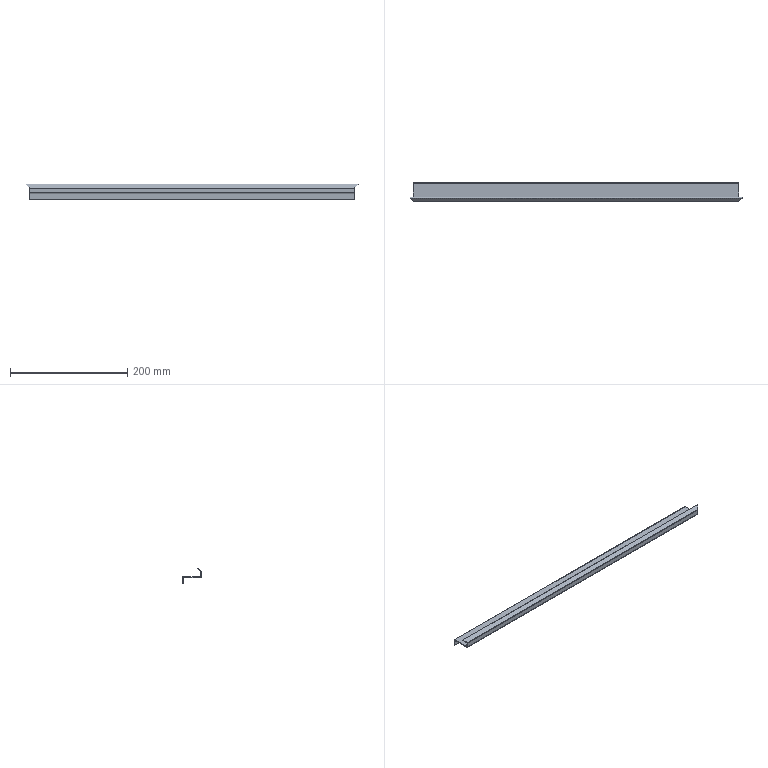Component | SolidWorks | UpperBeam-1 | 1 solid | 30 faces | box 566.33 x 32 x 26.16 mm | volume 48106 mm3 | plane 22 | cylinder 6 | spline 2 | commonest cylinder face diameters 3.2 x3 0.2 x3
STEP:
#1=COLOUR_RGB('',0.7922,0.8196,0.9333);
#2=FILL_AREA_STYLE_COLOUR('',#1);
#3=FILL_AREA_STYLE('',(#2));
#4=SURFACE_STYLE_FILL_AREA(#3);
#5=SURFACE_SIDE_STYLE('',(#4));
#6=SURFACE_STYLE_USAGE(.BOTH.,#5);
#7=PRESENTATION_STYLE_ASSIGNMENT((#6));
#8=CARTESIAN_POINT('',(9.198,12.971,37.604));
#9=VERTEX_POINT('',#8);
#10=CARTESIAN_POINT('',(9.198,14.105,37.604));
#11=VERTEX_POINT('',#10);
#12=CARTESIAN_POINT('',(9.198,12.908,37.604));
#13=DIRECTION('',(0.,1.,0.));
#14=VECTOR('',#13,39.37);
#15=LINE('',#12,#14);
#16=EDGE_CURVE('',#9,#11,#15,.T.);
#17=ORIENTED_EDGE('',*,*,#16,.T.);
#18=CARTESIAN_POINT('',(9.198,14.105,37.663));
#19=VERTEX_POINT('',#18);
#20=CARTESIAN_POINT('',(9.198,14.105,37.604));
#21=DIRECTION('',(0.,0.,1.));
#22=VECTOR('',#21,39.37);
#23=LINE('',#20,#22);
#24=EDGE_CURVE('',#11,#19,#23,.T.);
#25=ORIENTED_EDGE('',*,*,#24,.T.);
#26=CARTESIAN_POINT('',(9.198,12.971,37.663));
#27=VERTEX_POINT('',#26);
#28=CARTESIAN_POINT('',(9.198,12.908,37.663));
#29=DIRECTION('',(0.,1.,0.));
#30=VECTOR('',#29,39.37);
#31=LINE('',#28,#30);
#32=EDGE_CURVE('',#27,#19,#31,.T.);
#33=ORIENTED_EDGE('',*,*,#32,.F.);
#34=CARTESIAN_POINT('',(9.198,12.971,37.663));
#35=DIRECTION('',(0.,0.,-1.));
#36=VECTOR('',#35,39.37);
#37=LINE('',#34,#36);
#38=EDGE_CURVE('',#27,#9,#37,.T.);
#39=ORIENTED_EDGE('',*,*,#38,.T.);
#40=EDGE_LOOP('',(#17,#25,#33,#39));
#41=FACE_OUTER_BOUND('',#40,.T.);
#42=CARTESIAN_POINT('',(9.198,12.908,37.604));
#43=DIRECTION('',(1.,0.,0.));
#44=DIRECTION('',(0.,0.,-1.));
#45=AXIS2_PLACEMENT_3D('',#42,#43,#44);
#46=PLANE('',#45);
#47=ADVANCED_FACE('',(#41),#46,.T.);
#48=CARTESIAN_POINT('',(-12.691,14.105,37.604));
#49=VERTEX_POINT('',#48);
#50=CARTESIAN_POINT('',(-12.691,12.971,37.604));
#51=VERTEX_POINT('',#50);
#52=CARTESIAN_POINT('',(-12.691,12.908,37.604));
#53=DIRECTION('',(0.,-1.,0.));
#54=VECTOR('',#53,39.37);
#55=LINE('',#52,#54);
#56=EDGE_CURVE('',#49,#51,#55,.T.);
#57=ORIENTED_EDGE('',*,*,#56,.F.);
#58=CARTESIAN_POINT('',(9.198,14.105,37.604));
#59=DIRECTION('',(-1.,0.,0.));
#60=VECTOR('',#59,39.37);
#61=LINE('',#58,#60);
#62=EDGE_CURVE('',#11,#49,#61,.T.);
#63=ORIENTED_EDGE('',*,*,#62,.F.);
#64=ORIENTED_EDGE('',*,*,#16,.F.);
#65=CARTESIAN_POINT('',(9.198,12.971,37.604));
#66=DIRECTION('',(-1.,0.,0.));
#67=VECTOR('',#66,39.37);
#68=LINE('',#65,#67);
#69=EDGE_CURVE('',#9,#51,#68,.T.);
#70=ORIENTED_EDGE('',*,*,#69,.T.);
#71=EDGE_LOOP('',(#57,#63,#64,#70));
#72=FACE_OUTER_BOUND('',#71,.T.);
#73=CARTESIAN_POINT('',(-1.746,13.538,37.604));
#74=DIRECTION('',(0.,0.,-1.));
#75=DIRECTION('',(-1.,0.,0.));
#76=AXIS2_PLACEMENT_3D('',#73,#74,#75);
#77=PLANE('',#76);
#78=ADVANCED_FACE('',(#72),#77,.T.);
#79=CARTESIAN_POINT('',(-12.691,14.105,37.663));
#80=VERTEX_POINT('',#79);
#81=CARTESIAN_POINT('',(9.198,14.105,37.663));
#82=DIRECTION('',(-1.,0.,0.));
#83=VECTOR('',#82,39.37);
#84=LINE('',#81,#83);
#85=EDGE_CURVE('',#19,#80,#84,.T.);
#86=ORIENTED_EDGE('',*,*,#85,.T.);
#87=CARTESIAN_POINT('',(-12.691,12.971,37.663));
#88=VERTEX_POINT('',#87);
#89=CARTESIAN_POINT('',(-12.691,12.908,37.663));
#90=DIRECTION('',(0.,-1.,0.));
#91=VECTOR('',#90,39.37);
#92=LINE('',#89,#91);
#93=EDGE_CURVE('',#80,#88,#92,.T.);
#94=ORIENTED_EDGE('',*,*,#93,.T.);
#95=CARTESIAN_POINT('',(9.198,12.971,37.663));
#96=DIRECTION('',(-1.,0.,0.));
#97=VECTOR('',#96,39.37);
#98=LINE('',#95,#97);
#99=EDGE_CURVE('',#27,#88,#98,.T.);
#100=ORIENTED_EDGE('',*,*,#99,.F.);
#101=ORIENTED_EDGE('',*,*,#32,.T.);
#102=EDGE_LOOP('',(#86,#94,#100,#101));
#103=FACE_OUTER_BOUND('',#102,.T.);
#104=CARTESIAN_POINT('',(-1.746,13.538,37.663));
#105=DIRECTION('',(0.,0.,-1.));
#106=DIRECTION('',(-1.,0.,0.));
#107=AXIS2_PLACEMENT_3D('',#104,#105,#106);
#108=PLANE('',#107);
#109=ADVANCED_FACE('',(#103),#108,.F.);
#110=CARTESIAN_POINT('',(9.198,12.967,37.971));
#111=VERTEX_POINT('',#110);
#112=CARTESIAN_POINT('',(9.198,12.908,37.971));
#113=VERTEX_POINT('',#112);
#114=CARTESIAN_POINT('',(9.198,12.967,37.971));
#115=DIRECTION('',(0.,-1.,0.));
#116=VECTOR('',#115,39.37);
#117=LINE('',#114,#116);
#118=EDGE_CURVE('',#111,#113,#117,.T.);
#119=ORIENTED_EDGE('',*,*,#118,.T.);
#120=CARTESIAN_POINT('',(9.198,12.908,37.667));
#121=VERTEX_POINT('',#120);
#122=CARTESIAN_POINT('',(9.198,12.908,37.663));
#123=DIRECTION('',(0.,-0.,1.));
#124=VECTOR('',#123,39.37);
#125=LINE('',#122,#124);
#126=EDGE_CURVE('',#121,#113,#125,.T.);
#127=ORIENTED_EDGE('',*,*,#126,.F.);
#128=CARTESIAN_POINT('',(9.198,12.967,37.667));
#129=VERTEX_POINT('',#128);
#130=CARTESIAN_POINT('',(9.198,12.967,37.667));
#131=DIRECTION('',(0.,-1.,-0.));
#132=VECTOR('',#131,39.37);
#133=LINE('',#130,#132);
#134=EDGE_CURVE('',#129,#121,#133,.T.);
#135=ORIENTED_EDGE('',*,*,#134,.F.);
#136=CARTESIAN_POINT('',(9.198,12.967,37.998));
#137=DIRECTION('',(0.,-0.,1.));
#138=VECTOR('',#137,39.37);
#139=LINE('',#136,#138);
#140=EDGE_CURVE('',#129,#111,#139,.T.);
#141=ORIENTED_EDGE('',*,*,#140,.T.);
#142=EDGE_LOOP('',(#119,#127,#135,#141));
#143=FACE_OUTER_BOUND('',#142,.T.);
#144=CARTESIAN_POINT('',(9.198,12.908,37.998));
#145=DIRECTION('',(-1.,0.,0.));
#146=DIRECTION('',(0.,0.,1.));
#147=AXIS2_PLACEMENT_3D('',#144,#145,#146);
#148=PLANE('',#147);
#149=ADVANCED_FACE('',(#143),#148,.F.);
#150=CARTESIAN_POINT('',(-12.691,12.967,37.971));
#151=VERTEX_POINT('',#150);
#152=CARTESIAN_POINT('',(-12.691,12.908,37.971));
#153=VERTEX_POINT('',#152);
#154=CARTESIAN_POINT('',(-12.691,12.967,37.971));
#155=DIRECTION('',(0.,-1.,0.));
#156=VECTOR('',#155,39.37);
#157=LINE('',#154,#156);
#158=EDGE_CURVE('',#151,#153,#157,.T.);
#159=ORIENTED_EDGE('',*,*,#158,.F.);
#160=CARTESIAN_POINT('',(-12.691,12.967,37.667));
#161=VERTEX_POINT('',#160);
#162=CARTESIAN_POINT('',(-12.691,12.967,37.663));
#163=DIRECTION('',(0.,0.,-1.));
#164=VECTOR('',#163,39.37);
#165=LINE('',#162,#164);
#166=EDGE_CURVE('',#151,#161,#165,.T.);
#167=ORIENTED_EDGE('',*,*,#166,.T.);
#168=CARTESIAN_POINT('',(-12.691,12.908,37.667));
#169=VERTEX_POINT('',#168);
#170=CARTESIAN_POINT('',(-12.691,12.908,37.667));
#171=DIRECTION('',(0.,-1.,-0.));
#172=VECTOR('',#171,39.37);
#173=LINE('',#170,#172);
#174=EDGE_CURVE('',#161,#169,#173,.T.);
#175=ORIENTED_EDGE('',*,*,#174,.T.);
#176=CARTESIAN_POINT('',(-12.691,12.908,37.663));
#177=DIRECTION('',(0.,0.,-1.));
#178=VECTOR('',#177,39.37);
#179=LINE('',#176,#178);
#180=EDGE_CURVE('',#153,#169,#179,.T.);
#181=ORIENTED_EDGE('',*,*,#180,.F.);
#182=EDGE_LOOP('',(#159,#167,#175,#181));
#183=FACE_OUTER_BOUND('',#182,.T.);
#184=CARTESIAN_POINT('',(-12.691,12.908,37.663));
#185=DIRECTION('',(1.,0.,0.));
#186=DIRECTION('',(0.,0.,-1.));
#187=AXIS2_PLACEMENT_3D('',#184,#185,#186);
#188=PLANE('',#187);
#189=ADVANCED_FACE('',(#183),#188,.F.);
#190=CARTESIAN_POINT('',(9.2,12.908,37.971));
#191=DIRECTION('',(-1.,0.,0.));
#192=VECTOR('',#191,39.37);
#193=LINE('',#190,#192);
#194=EDGE_CURVE('',#113,#153,#193,.T.);
#195=ORIENTED_EDGE('',*,*,#194,.T.);
#196=ORIENTED_EDGE('',*,*,#180,.T.);
#197=CARTESIAN_POINT('',(-12.691,12.908,37.667));
#198=DIRECTION('',(-1.,-0.,0.));
#199=VECTOR('',#198,39.37);
#200=LINE('',#197,#199);
#201=EDGE_CURVE('',#121,#169,#200,.T.);
#202=ORIENTED_EDGE('',*,*,#201,.F.);
#203=ORIENTED_EDGE('',*,*,#126,.T.);
#204=EDGE_LOOP('',(#195,#196,#202,#203));
#205=FACE_OUTER_BOUND('',#204,.T.);
#206=CARTESIAN_POINT('',(-1.746,12.908,37.663));
#207=DIRECTION('',(0.,1.,0.));
#208=DIRECTION('',(0.,-0.,1.));
#209=AXIS2_PLACEMENT_3D('',#206,#207,#208);
#210=PLANE('',#209);
#211=ADVANCED_FACE('',(#205),#210,.F.);
#212=ORIENTED_EDGE('',*,*,#166,.F.);
#213=CARTESIAN_POINT('',(9.2,12.967,37.971));
#214=DIRECTION('',(-1.,0.,0.));
#215=VECTOR('',#214,39.37);
#216=LINE('',#213,#215);
#217=EDGE_CURVE('',#111,#151,#216,.T.);
#218=ORIENTED_EDGE('',*,*,#217,.F.);
#219=ORIENTED_EDGE('',*,*,#140,.F.);
#220=CARTESIAN_POINT('',(-12.691,12.967,37.667));
#221=DIRECTION('',(1.,0.,-0.));
#222=VECTOR('',#221,39.37);
#223=LINE('',#220,#222);
#224=EDGE_CURVE('',#161,#129,#223,.T.);
#225=ORIENTED_EDGE('',*,*,#224,.F.);
#226=EDGE_LOOP('',(#212,#218,#219,#225));
#227=FACE_OUTER_BOUND('',#226,.T.);
#228=CARTESIAN_POINT('',(-1.746,12.967,37.663));
#229=DIRECTION('',(0.,1.,0.));
#230=DIRECTION('',(0.,-0.,1.));
#231=AXIS2_PLACEMENT_3D('',#228,#229,#230);
#232=PLANE('',#231);
#233=ADVANCED_FACE('',(#227),#232,.T.);
#234=CARTESIAN_POINT('',(-12.691,14.105,37.604));
#235=DIRECTION('',(0.,0.,1.));
#236=VECTOR('',#235,39.37);
#237=LINE('',#234,#236);
#238=EDGE_CURVE('',#49,#80,#237,.T.);
#239=ORIENTED_EDGE('',*,*,#238,.F.);
#240=ORIENTED_EDGE('',*,*,#56,.T.);
#241=CARTESIAN_POINT('',(-12.691,12.971,37.663));
#242=DIRECTION('',(0.,0.,-1.));
#243=VECTOR('',#242,39.37);
#244=LINE('',#241,#243);
#245=EDGE_CURVE('',#88,#51,#244,.T.);
#246=ORIENTED_EDGE('',*,*,#245,.F.);
#247=ORIENTED_EDGE('',*,*,#93,.F.);
#248=EDGE_LOOP('',(#239,#240,#246,#247));
#249=FACE_OUTER_BOUND('',#248,.T.);
#250=CARTESIAN_POINT('',(-12.691,12.908,37.604));
#251=DIRECTION('',(-1.,0.,0.));
#252=DIRECTION('',(0.,0.,1.));
#253=AXIS2_PLACEMENT_3D('',#250,#251,#252);
#254=PLANE('',#253);
#255=ADVANCED_FACE('',(#249),#254,.T.);
#256=ORIENTED_EDGE('',*,*,#174,.F.);
#257=CARTESIAN_POINT('',(-12.691,12.971,37.667));
#258=DIRECTION('',(-1.,0.,0.));
#259=DIRECTION('',(0.,0.,-1.));
#260=AXIS2_PLACEMENT_3D('',#257,#258,#259);
#261=CIRCLE('',#260,0.003937);
#262=EDGE_CURVE('',#88,#161,#261,.T.);
#263=ORIENTED_EDGE('',*,*,#262,.F.);
#264=ORIENTED_EDGE('',*,*,#245,.T.);
#265=CARTESIAN_POINT('',(-12.691,12.971,37.667));
#266=DIRECTION('',(-1.,0.,0.));
#267=DIRECTION('',(0.,0.,-1.));
#268=AXIS2_PLACEMENT_3D('',#265,#266,#267);
#269=CIRCLE('',#268,0.06299);
#270=EDGE_CURVE('',#51,#169,#269,.T.);
#271=ORIENTED_EDGE('',*,*,#270,.T.);
#272=EDGE_LOOP('',(#256,#263,#264,#271));
#273=FACE_OUTER_BOUND('',#272,.T.);
#274=CARTESIAN_POINT('',(-12.691,12.971,37.667));
#275=DIRECTION('',(-1.,0.,0.));
#276=DIRECTION('',(0.,0.,1.));
#277=AXIS2_PLACEMENT_3D('',#274,#275,#276);
#278=PLANE('',#277);
#279=ADVANCED_FACE('',(#273),#278,.T.);
#280=CARTESIAN_POINT('',(9.198,12.971,37.667));
#281=DIRECTION('',(1.,0.,0.));
#282=DIRECTION('',(0.,0.,-1.));
#283=AXIS2_PLACEMENT_3D('',#280,#281,#282);
#284=CIRCLE('',#283,0.003937);
#285=EDGE_CURVE('',#129,#27,#284,.T.);
#286=ORIENTED_EDGE('',*,*,#285,.F.);
#287=ORIENTED_EDGE('',*,*,#134,.T.);
#288=CARTESIAN_POINT('',(9.198,12.971,37.667));
#289=DIRECTION('',(1.,0.,0.));
#290=DIRECTION('',(0.,0.,-1.));
#291=AXIS2_PLACEMENT_3D('',#288,#289,#290);
#292=CIRCLE('',#291,0.06299);
#293=EDGE_CURVE('',#121,#9,#292,.T.);
#294=ORIENTED_EDGE('',*,*,#293,.T.);
#295=ORIENTED_EDGE('',*,*,#38,.F.);
#296=EDGE_LOOP('',(#286,#287,#294,#295));
#297=FACE_OUTER_BOUND('',#296,.T.);
#298=CARTESIAN_POINT('',(9.198,12.971,37.667));
#299=DIRECTION('',(-1.,0.,0.));
#300=DIRECTION('',(0.,0.,1.));
#301=AXIS2_PLACEMENT_3D('',#298,#299,#300);
#302=PLANE('',#301);
#303=ADVANCED_FACE('',(#297),#302,.F.);
#304=ORIENTED_EDGE('',*,*,#69,.F.);
#305=ORIENTED_EDGE('',*,*,#293,.F.);
#306=ORIENTED_EDGE('',*,*,#201,.T.);
#307=ORIENTED_EDGE('',*,*,#270,.F.);
#308=EDGE_LOOP('',(#304,#305,#306,#307));
#309=FACE_OUTER_BOUND('',#308,.T.);
#310=CARTESIAN_POINT('',(9.198,12.971,37.667));
#311=DIRECTION('',(1.,0.,0.));
#312=DIRECTION('',(0.,-1.,0.));
#313=AXIS2_PLACEMENT_3D('',#310,#311,#312);
#314=CYLINDRICAL_SURFACE('',#313,0.06299);
#315=ADVANCED_FACE('',(#309),#314,.T.);
#316=ORIENTED_EDGE('',*,*,#99,.T.);
#317=ORIENTED_EDGE('',*,*,#262,.T.);
#318=ORIENTED_EDGE('',*,*,#224,.T.);
#319=ORIENTED_EDGE('',*,*,#285,.T.);
#320=EDGE_LOOP('',(#316,#317,#318,#319));
#321=FACE_OUTER_BOUND('',#320,.T.);
#322=CARTESIAN_POINT('',(9.198,12.971,37.667));
#323=DIRECTION('',(1.,0.,0.));
#324=DIRECTION('',(0.,-1.,0.));
#325=AXIS2_PLACEMENT_3D('',#322,#323,#324);
#326=CYLINDRICAL_SURFACE('',#325,0.003937);
#327=ADVANCED_FACE('',(#321),#326,.F.);
#328=CARTESIAN_POINT('',(-12.692,12.968,37.974));
#329=VERTEX_POINT('',#328);
#330=CARTESIAN_POINT('',(-12.692,12.927,38.016));
#331=VERTEX_POINT('',#330);
#332=CARTESIAN_POINT('',(-12.692,12.927,38.016));
#333=DIRECTION('',(0.,-0.7071,0.7071));
#334=VECTOR('',#333,39.37);
#335=LINE('',#332,#334);
#336=EDGE_CURVE('',#329,#331,#335,.T.);
#337=ORIENTED_EDGE('',*,*,#336,.F.);
#338=CARTESIAN_POINT('',(-12.691,12.967,37.971));
#339=CARTESIAN_POINT('',(-12.692,12.967,37.972));
#340=CARTESIAN_POINT('',(-12.692,12.968,37.973));
#341=CARTESIAN_POINT('',(-12.692,12.968,37.974));
#342=B_SPLINE_CURVE_WITH_KNOTS('',3,(#338,#339,#340,#341),.UNSPECIFIED.,.F.,.F.,(4,4),(0.,1.),.UNSPECIFIED.);
#343=EDGE_CURVE('',#151,#329,#342,.T.);
#344=ORIENTED_EDGE('',*,*,#343,.F.);
#345=ORIENTED_EDGE('',*,*,#158,.T.);
#346=CARTESIAN_POINT('',(-12.691,12.908,37.971));
#347=CARTESIAN_POINT('',(-12.692,12.908,37.98));
#348=CARTESIAN_POINT('',(-12.692,12.91,37.988));
#349=CARTESIAN_POINT('',(-12.692,12.916,38.003));
#350=CARTESIAN_POINT('',(-12.692,12.921,38.01));
#351=CARTESIAN_POINT('',(-12.692,12.927,38.016));
#352=B_SPLINE_CURVE_WITH_KNOTS('',3,(#346,#347,#348,#349,#350,#351),.UNSPECIFIED.,.F.,.F.,(4,2,4),(0.,0.5,1.),.UNSPECIFIED.);
#353=EDGE_CURVE('',#153,#331,#352,.T.);
#354=ORIENTED_EDGE('',*,*,#353,.T.);
#355=EDGE_LOOP('',(#337,#344,#345,#354));
#356=FACE_OUTER_BOUND('',#355,.T.);
#357=CARTESIAN_POINT('',(-12.691,12.908,37.971));
#358=CARTESIAN_POINT('',(-12.692,12.908,37.98));
#359=CARTESIAN_POINT('',(-12.692,12.909,37.988));
#360=CARTESIAN_POINT('',(-12.692,12.916,38.003));
#361=CARTESIAN_POINT('',(-12.692,12.92,38.011));
#362=CARTESIAN_POINT('',(-12.692,12.926,38.016));
#363=CARTESIAN_POINT('',(-12.691,12.908,37.971));
#364=CARTESIAN_POINT('',(-12.692,12.908,37.98));
#365=CARTESIAN_POINT('',(-12.692,12.91,37.988));
#366=CARTESIAN_POINT('',(-12.692,12.916,38.003));
#367=CARTESIAN_POINT('',(-12.692,12.921,38.01));
#368=CARTESIAN_POINT('',(-12.692,12.927,38.016));
#369=CARTESIAN_POINT('',(-12.691,12.967,37.971));
#370=CARTESIAN_POINT('',(-12.692,12.967,37.972));
#371=CARTESIAN_POINT('',(-12.692,12.967,37.972));
#372=CARTESIAN_POINT('',(-12.692,12.968,37.973));
#373=CARTESIAN_POINT('',(-12.692,12.968,37.974));
#374=CARTESIAN_POINT('',(-12.692,12.968,37.974));
#375=B_SPLINE_SURFACE_WITH_KNOTS('',1,3,((#357,#358,#359,#360,#361,#362),(#363,#364,#365,#366,#367,#368),(#369,#370,#371,#372,#373,#374)),.UNSPECIFIED.,.F.,.F.,.F.,(2,1,2),(4,2,4),(-0.01,0.,1.),(0.,0.5,1.),.UNSPECIFIED.);
#376=ADVANCED_FACE('',(#356),#375,.F.);
#377=CARTESIAN_POINT('',(9.2,12.968,37.974));
#378=VERTEX_POINT('',#377);
#379=CARTESIAN_POINT('',(9.2,12.968,37.974));
#380=CARTESIAN_POINT('',(9.199,12.968,37.973));
#381=CARTESIAN_POINT('',(9.199,12.967,37.972));
#382=CARTESIAN_POINT('',(9.198,12.967,37.971));
#383=B_SPLINE_CURVE_WITH_KNOTS('',3,(#379,#380,#381,#382),.UNSPECIFIED.,.F.,.F.,(4,4),(0.,1.),.UNSPECIFIED.);
#384=EDGE_CURVE('',#378,#111,#383,.T.);
#385=ORIENTED_EDGE('',*,*,#384,.F.);
#386=CARTESIAN_POINT('',(9.2,12.927,38.016));
#387=VERTEX_POINT('',#386);
#388=CARTESIAN_POINT('',(9.2,12.968,37.974));
#389=DIRECTION('',(-0.,-0.7071,0.7071));
#390=VECTOR('',#389,39.37);
#391=LINE('',#388,#390);
#392=EDGE_CURVE('',#378,#387,#391,.T.);
#393=ORIENTED_EDGE('',*,*,#392,.T.);
#394=CARTESIAN_POINT('',(9.2,12.927,38.016));
#395=CARTESIAN_POINT('',(9.199,12.921,38.01));
#396=CARTESIAN_POINT('',(9.199,12.916,38.003));
#397=CARTESIAN_POINT('',(9.199,12.91,37.988));
#398=CARTESIAN_POINT('',(9.199,12.908,37.98));
#399=CARTESIAN_POINT('',(9.198,12.908,37.971));
#400=B_SPLINE_CURVE_WITH_KNOTS('',3,(#394,#395,#396,#397,#398,#399),.UNSPECIFIED.,.F.,.F.,(4,2,4),(0.,0.5,1.),.UNSPECIFIED.);
#401=EDGE_CURVE('',#387,#113,#400,.T.);
#402=ORIENTED_EDGE('',*,*,#401,.T.);
#403=ORIENTED_EDGE('',*,*,#118,.F.);
#404=EDGE_LOOP('',(#385,#393,#402,#403));
#405=FACE_OUTER_BOUND('',#404,.T.);
#406=CARTESIAN_POINT('',(9.2,12.926,38.016));
#407=CARTESIAN_POINT('',(9.199,12.92,38.011));
#408=CARTESIAN_POINT('',(9.199,12.916,38.003));
#409=CARTESIAN_POINT('',(9.199,12.909,37.988));
#410=CARTESIAN_POINT('',(9.199,12.908,37.98));
#411=CARTESIAN_POINT('',(9.198,12.908,37.971));
#412=CARTESIAN_POINT('',(9.2,12.927,38.016));
#413=CARTESIAN_POINT('',(9.199,12.921,38.01));
#414=CARTESIAN_POINT('',(9.199,12.916,38.003));
#415=CARTESIAN_POINT('',(9.199,12.91,37.988));
#416=CARTESIAN_POINT('',(9.199,12.908,37.98));
#417=CARTESIAN_POINT('',(9.198,12.908,37.971));
#418=CARTESIAN_POINT('',(9.2,12.968,37.974));
#419=CARTESIAN_POINT('',(9.199,12.968,37.974));
#420=CARTESIAN_POINT('',(9.199,12.968,37.973));
#421=CARTESIAN_POINT('',(9.199,12.967,37.972));
#422=CARTESIAN_POINT('',(9.199,12.967,37.972));
#423=CARTESIAN_POINT('',(9.198,12.967,37.971));
#424=B_SPLINE_SURFACE_WITH_KNOTS('',1,3,((#406,#407,#408,#409,#410,#411),(#412,#413,#414,#415,#416,#417),(#418,#419,#420,#421,#422,#423)),.UNSPECIFIED.,.F.,.F.,.F.,(2,1,2),(4,2,4),(-0.01,0.,1.),(0.,0.5,1.),.UNSPECIFIED.);
#425=ADVANCED_FACE('',(#405),#424,.F.);
#426=ORIENTED_EDGE('',*,*,#194,.F.);
#427=ORIENTED_EDGE('',*,*,#401,.F.);
#428=CARTESIAN_POINT('',(-12.692,12.927,38.016));
#429=DIRECTION('',(-1.,-0.,-0.));
#430=VECTOR('',#429,39.37);
#431=LINE('',#428,#430);
#432=EDGE_CURVE('',#387,#331,#431,.T.);
#433=ORIENTED_EDGE('',*,*,#432,.T.);
#434=ORIENTED_EDGE('',*,*,#353,.F.);
#435=EDGE_LOOP('',(#426,#427,#433,#434));
#436=FACE_OUTER_BOUND('',#435,.T.);
#437=CARTESIAN_POINT('',(9.2,12.971,37.971));
#438=DIRECTION('',(1.,0.,0.));
#439=DIRECTION('',(0.,-0.7071,0.7071));
#440=AXIS2_PLACEMENT_3D('',#437,#438,#439);
#441=CYLINDRICAL_SURFACE('',#440,0.06299);
#442=ADVANCED_FACE('',(#436),#441,.T.);
#443=ORIENTED_EDGE('',*,*,#217,.T.);
#444=ORIENTED_EDGE('',*,*,#343,.T.);
#445=CARTESIAN_POINT('',(-12.692,12.968,37.974));
#446=DIRECTION('',(1.,0.,0.));
#447=VECTOR('',#446,39.37);
#448=LINE('',#445,#447);
#449=EDGE_CURVE('',#329,#378,#448,.T.);
#450=ORIENTED_EDGE('',*,*,#449,.T.);
#451=ORIENTED_EDGE('',*,*,#384,.T.);
#452=EDGE_LOOP('',(#443,#444,#450,#451));
#453=FACE_OUTER_BOUND('',#452,.T.);
#454=CARTESIAN_POINT('',(9.2,12.971,37.971));
#455=DIRECTION('',(1.,0.,0.));
#456=DIRECTION('',(0.,-0.7071,0.7071));
#457=AXIS2_PLACEMENT_3D('',#454,#455,#456);
#458=CYLINDRICAL_SURFACE('',#457,0.003937);
#459=ADVANCED_FACE('',(#453),#458,.F.);
#460=ORIENTED_EDGE('',*,*,#392,.F.);
#461=CARTESIAN_POINT('',(9.402,13.173,38.178));
#462=VERTEX_POINT('',#461);
#463=CARTESIAN_POINT('',(9.402,13.173,38.178));
#464=DIRECTION('',(0.5736,0.5792,0.5792));
#465=VECTOR('',#464,39.37);
#466=LINE('',#463,#465);
#467=EDGE_CURVE('',#378,#462,#466,.T.);
#468=ORIENTED_EDGE('',*,*,#467,.T.);
#469=CARTESIAN_POINT('',(9.402,13.131,38.22));
#470=VERTEX_POINT('',#469);
#471=CARTESIAN_POINT('',(9.402,13.131,38.22));
#472=DIRECTION('',(0.,0.7071,-0.7071));
#473=VECTOR('',#472,39.37);
#474=LINE('',#471,#473);
#475=EDGE_CURVE('',#470,#462,#474,.T.);
#476=ORIENTED_EDGE('',*,*,#475,.F.);
#477=CARTESIAN_POINT('',(5.676,9.369,34.458));
#478=DIRECTION('',(0.5736,0.5792,0.5792));
#479=VECTOR('',#478,39.37);
#480=LINE('',#477,#479);
#481=EDGE_CURVE('',#387,#470,#480,.T.);
#482=ORIENTED_EDGE('',*,*,#481,.F.);
#483=EDGE_LOOP('',(#460,#468,#476,#482));
#484=FACE_OUTER_BOUND('',#483,.T.);
#485=CARTESIAN_POINT('',(9.402,13.131,38.22));
#486=DIRECTION('',(-0.8192,0.4056,0.4056));
#487=DIRECTION('',(0.4437,0.,0.8962));
#488=AXIS2_PLACEMENT_3D('',#485,#486,#487);
#489=PLANE('',#488);
#490=ADVANCED_FACE('',(#484),#489,.F.);
#491=ORIENTED_EDGE('',*,*,#336,.T.);
#492=CARTESIAN_POINT('',(-12.895,13.131,38.22));
#493=VERTEX_POINT('',#492);
#494=CARTESIAN_POINT('',(-9.169,9.369,34.458));
#495=DIRECTION('',(0.5736,-0.5792,-0.5792));
#496=VECTOR('',#495,39.37);
#497=LINE('',#494,#496);
#498=EDGE_CURVE('',#493,#331,#497,.T.);
#499=ORIENTED_EDGE('',*,*,#498,.F.);
#500=CARTESIAN_POINT('',(-12.895,13.173,38.178));
#501=VERTEX_POINT('',#500);
#502=CARTESIAN_POINT('',(-12.895,13.131,38.22));
#503=DIRECTION('',(-0.,0.7071,-0.7071));
#504=VECTOR('',#503,39.37);
#505=LINE('',#502,#504);
#506=EDGE_CURVE('',#493,#501,#505,.T.);
#507=ORIENTED_EDGE('',*,*,#506,.T.);
#508=CARTESIAN_POINT('',(-12.691,12.967,37.973));
#509=DIRECTION('',(0.5736,-0.5792,-0.5792));
#510=VECTOR('',#509,39.37);
#511=LINE('',#508,#510);
#512=EDGE_CURVE('',#501,#329,#511,.T.);
#513=ORIENTED_EDGE('',*,*,#512,.T.);
#514=EDGE_LOOP('',(#491,#499,#507,#513));
#515=FACE_OUTER_BOUND('',#514,.T.);
#516=CARTESIAN_POINT('',(-12.691,12.926,38.015));
#517=DIRECTION('',(0.8192,0.4056,0.4056));
#518=DIRECTION('',(0.4437,0.,-0.8962));
#519=AXIS2_PLACEMENT_3D('',#516,#517,#518);
#520=PLANE('',#519);
#521=ADVANCED_FACE('',(#515),#520,.F.);
#522=ORIENTED_EDGE('',*,*,#432,.F.);
#523=ORIENTED_EDGE('',*,*,#481,.T.);
#524=CARTESIAN_POINT('',(-1.746,13.131,38.22));
#525=DIRECTION('',(-1.,0.,0.));
#526=VECTOR('',#525,39.37);
#527=LINE('',#524,#526);
#528=EDGE_CURVE('',#470,#493,#527,.T.);
#529=ORIENTED_EDGE('',*,*,#528,.T.);
#530=ORIENTED_EDGE('',*,*,#498,.T.);
#531=EDGE_LOOP('',(#522,#523,#529,#530));
#532=FACE_OUTER_BOUND('',#531,.T.);
#533=CARTESIAN_POINT('',(-1.746,13.044,38.133));
#534=DIRECTION('',(0.,0.7071,-0.7071));
#535=DIRECTION('',(0.,0.7071,0.7071));
#536=AXIS2_PLACEMENT_3D('',#533,#534,#535);
#537=PLANE('',#536);
#538=ADVANCED_FACE('',(#532),#537,.F.);
#539=ORIENTED_EDGE('',*,*,#467,.F.);
#540=ORIENTED_EDGE('',*,*,#449,.F.);
#541=ORIENTED_EDGE('',*,*,#512,.F.);
#542=CARTESIAN_POINT('',(-12.895,13.173,38.178));
#543=DIRECTION('',(-1.,0.,0.));
#544=VECTOR('',#543,39.37);
#545=LINE('',#542,#544);
#546=EDGE_CURVE('',#462,#501,#545,.T.);
#547=ORIENTED_EDGE('',*,*,#546,.F.);
#548=EDGE_LOOP('',(#539,#540,#541,#547));
#549=FACE_OUTER_BOUND('',#548,.T.);
#550=CARTESIAN_POINT('',(-1.746,13.085,38.091));
#551=DIRECTION('',(0.,0.7071,-0.7071));
#552=DIRECTION('',(0.,0.7071,0.7071));
#553=AXIS2_PLACEMENT_3D('',#550,#551,#552);
#554=PLANE('',#553);
#555=ADVANCED_FACE('',(#549),#554,.T.);
#556=ORIENTED_EDGE('',*,*,#546,.T.);
#557=ORIENTED_EDGE('',*,*,#506,.F.);
#558=ORIENTED_EDGE('',*,*,#528,.F.);
#559=ORIENTED_EDGE('',*,*,#475,.T.);
#560=EDGE_LOOP('',(#556,#557,#558,#559));
#561=FACE_OUTER_BOUND('',#560,.T.);
#562=CARTESIAN_POINT('',(-12.895,13.131,38.22));
#563=DIRECTION('',(0.,-0.7071,-0.7071));
#564=DIRECTION('',(0.,0.7071,-0.7071));
#565=AXIS2_PLACEMENT_3D('',#562,#563,#564);
#566=PLANE('',#565);
#567=ADVANCED_FACE('',(#561),#566,.F.);
#568=CARTESIAN_POINT('',(-12.691,14.109,37.6));
#569=VERTEX_POINT('',#568);
#570=CARTESIAN_POINT('',(-12.691,14.168,37.6));
#571=VERTEX_POINT('',#570);
#572=CARTESIAN_POINT('',(-12.691,14.168,37.6));
#573=DIRECTION('',(0.,1.,0.));
#574=VECTOR('',#573,39.37);
#575=LINE('',#572,#574);
#576=EDGE_CURVE('',#569,#571,#575,.T.);
#577=ORIENTED_EDGE('',*,*,#576,.F.);
#578=CARTESIAN_POINT('',(-12.691,14.105,37.6));
#579=DIRECTION('',(-1.,0.,0.));
#580=DIRECTION('',(0.,0.,-1.));
#581=AXIS2_PLACEMENT_3D('',#578,#579,#580);
#582=CIRCLE('',#581,0.003937);
#583=EDGE_CURVE('',#49,#569,#582,.T.);
#584=ORIENTED_EDGE('',*,*,#583,.F.);
#585=ORIENTED_EDGE('',*,*,#238,.T.);
#586=CARTESIAN_POINT('',(-12.691,14.105,37.6));
#587=DIRECTION('',(-1.,0.,0.));
#588=DIRECTION('',(0.,0.,-1.));
#589=AXIS2_PLACEMENT_3D('',#586,#587,#588);
#590=CIRCLE('',#589,0.06299);
#591=EDGE_CURVE('',#80,#571,#590,.T.);
#592=ORIENTED_EDGE('',*,*,#591,.T.);
#593=EDGE_LOOP('',(#577,#584,#585,#592));
#594=FACE_OUTER_BOUND('',#593,.T.);
#595=CARTESIAN_POINT('',(-12.691,14.105,37.6));
#596=DIRECTION('',(-1.,0.,0.));
#597=DIRECTION('',(0.,0.,1.));
#598=AXIS2_PLACEMENT_3D('',#595,#596,#597);
#599=PLANE('',#598);
#600=ADVANCED_FACE('',(#594),#599,.T.);
#601=CARTESIAN_POINT('',(9.198,14.109,37.6));
#602=VERTEX_POINT('',#601);
#603=CARTESIAN_POINT('',(9.198,14.105,37.6));
#604=DIRECTION('',(1.,0.,0.));
#605=DIRECTION('',(0.,0.,-1.));
#606=AXIS2_PLACEMENT_3D('',#603,#604,#605);
#607=CIRCLE('',#606,0.003937);
#608=EDGE_CURVE('',#602,#11,#607,.T.);
#609=ORIENTED_EDGE('',*,*,#608,.F.);
#610=CARTESIAN_POINT('',(9.198,14.168,37.6));
#611=VERTEX_POINT('',#610);
#612=CARTESIAN_POINT('',(9.198,14.109,37.6));
#613=DIRECTION('',(0.,1.,0.));
#614=VECTOR('',#613,39.37);
#615=LINE('',#612,#614);
#616=EDGE_CURVE('',#602,#611,#615,.T.);
#617=ORIENTED_EDGE('',*,*,#616,.T.);
#618=CARTESIAN_POINT('',(9.198,14.105,37.6));
#619=DIRECTION('',(1.,0.,0.));
#620=DIRECTION('',(0.,0.,-1.));
#621=AXIS2_PLACEMENT_3D('',#618,#619,#620);
#622=CIRCLE('',#621,0.06299);
#623=EDGE_CURVE('',#611,#19,#622,.T.);
#624=ORIENTED_EDGE('',*,*,#623,.T.);
#625=ORIENTED_EDGE('',*,*,#24,.F.);
#626=EDGE_LOOP('',(#609,#617,#624,#625));
#627=FACE_OUTER_BOUND('',#626,.T.);
#628=CARTESIAN_POINT('',(9.198,14.105,37.6));
#629=DIRECTION('',(-1.,0.,0.));
#630=DIRECTION('',(0.,0.,1.));
#631=AXIS2_PLACEMENT_3D('',#628,#629,#630);
#632=PLANE('',#631);
#633=ADVANCED_FACE('',(#627),#632,.F.);
#634=ORIENTED_EDGE('',*,*,#85,.F.);
#635=ORIENTED_EDGE('',*,*,#623,.F.);
#636=CARTESIAN_POINT('',(-12.691,14.168,37.6));
#637=DIRECTION('',(-1.,0.,-0.));
#638=VECTOR('',#637,39.37);
#639=LINE('',#636,#638);
#640=EDGE_CURVE('',#611,#571,#639,.T.);
#641=ORIENTED_EDGE('',*,*,#640,.T.);
#642=ORIENTED_EDGE('',*,*,#591,.F.);
#643=EDGE_LOOP('',(#634,#635,#641,#642));
#644=FACE_OUTER_BOUND('',#643,.T.);
#645=CARTESIAN_POINT('',(9.198,14.105,37.6));
#646=DIRECTION('',(1.,0.,0.));
#647=DIRECTION('',(0.,1.,0.));
#648=AXIS2_PLACEMENT_3D('',#645,#646,#647);
#649=CYLINDRICAL_SURFACE('',#648,0.06299);
#650=ADVANCED_FACE('',(#644),#649,.T.);
#651=ORIENTED_EDGE('',*,*,#62,.T.);
#652=ORIENTED_EDGE('',*,*,#583,.T.);
#653=CARTESIAN_POINT('',(-12.691,14.109,37.6));
#654=DIRECTION('',(1.,-0.,0.));
#655=VECTOR('',#654,39.37);
#656=LINE('',#653,#655);
#657=EDGE_CURVE('',#569,#602,#656,.T.);
#658=ORIENTED_EDGE('',*,*,#657,.T.);
#659=ORIENTED_EDGE('',*,*,#608,.T.);
#660=EDGE_LOOP('',(#651,#652,#658,#659));
#661=FACE_OUTER_BOUND('',#660,.T.);
#662=CARTESIAN_POINT('',(9.198,14.105,37.6));
#663=DIRECTION('',(1.,0.,0.));
#664=DIRECTION('',(0.,1.,0.));
#665=AXIS2_PLACEMENT_3D('',#662,#663,#664);
#666=CYLINDRICAL_SURFACE('',#665,0.003937);
#667=ADVANCED_FACE('',(#661),#666,.F.);
#668=ORIENTED_EDGE('',*,*,#616,.F.);
#669=CARTESIAN_POINT('',(9.198,14.109,37.19));
#670=VERTEX_POINT('',#669);
#671=CARTESIAN_POINT('',(9.198,14.109,37.19));
#672=DIRECTION('',(0.,0.,-1.));
#673=VECTOR('',#672,39.37);
#674=LINE('',#671,#673);
#675=EDGE_CURVE('',#602,#670,#674,.T.);
#676=ORIENTED_EDGE('',*,*,#675,.T.);
#677=CARTESIAN_POINT('',(9.198,14.168,37.19));
#678=VERTEX_POINT('',#677);
#679=CARTESIAN_POINT('',(9.198,14.168,37.19));
#680=DIRECTION('',(0.,-1.,-0.));
#681=VECTOR('',#680,39.37);
#682=LINE('',#679,#681);
#683=EDGE_CURVE('',#678,#670,#682,.T.);
#684=ORIENTED_EDGE('',*,*,#683,.F.);
#685=CARTESIAN_POINT('',(9.198,14.168,37.663));
#686=DIRECTION('',(0.,0.,-1.));
#687=VECTOR('',#686,39.37);
#688=LINE('',#685,#687);
#689=EDGE_CURVE('',#611,#678,#688,.T.);
#690=ORIENTED_EDGE('',*,*,#689,.F.);
#691=EDGE_LOOP('',(#668,#676,#684,#690));
#692=FACE_OUTER_BOUND('',#691,.T.);
#693=CARTESIAN_POINT('',(9.198,14.168,37.19));
#694=DIRECTION('',(-1.,0.,0.));
#695=DIRECTION('',(0.,0.,1.));
#696=AXIS2_PLACEMENT_3D('',#693,#694,#695);
#697=PLANE('',#696);
#698=ADVANCED_FACE('',(#692),#697,.F.);
#699=ORIENTED_EDGE('',*,*,#576,.T.);
#700=CARTESIAN_POINT('',(-12.691,14.168,37.19));
#701=VERTEX_POINT('',#700);
#702=CARTESIAN_POINT('',(-12.691,14.168,37.663));
#703=DIRECTION('',(0.,-0.,1.));
#704=VECTOR('',#703,39.37);
#705=LINE('',#702,#704);
#706=EDGE_CURVE('',#701,#571,#705,.T.);
#707=ORIENTED_EDGE('',*,*,#706,.F.);
#708=CARTESIAN_POINT('',(-12.691,14.109,37.19));
#709=VERTEX_POINT('',#708);
#710=CARTESIAN_POINT('',(-12.691,14.168,37.19));
#711=DIRECTION('',(0.,-1.,-0.));
#712=VECTOR('',#711,39.37);
#713=LINE('',#710,#712);
#714=EDGE_CURVE('',#701,#709,#713,.T.);
#715=ORIENTED_EDGE('',*,*,#714,.T.);
#716=CARTESIAN_POINT('',(-12.691,14.109,37.604));
#717=DIRECTION('',(0.,-0.,1.));
#718=VECTOR('',#717,39.37);
#719=LINE('',#716,#718);
#720=EDGE_CURVE('',#709,#569,#719,.T.);
#721=ORIENTED_EDGE('',*,*,#720,.T.);
#722=EDGE_LOOP('',(#699,#707,#715,#721));
#723=FACE_OUTER_BOUND('',#722,.T.);
#724=CARTESIAN_POINT('',(-12.691,14.168,37.604));
#725=DIRECTION('',(1.,0.,0.));
#726=DIRECTION('',(0.,0.,-1.));
#727=AXIS2_PLACEMENT_3D('',#724,#725,#726);
#728=PLANE('',#727);
#729=ADVANCED_FACE('',(#723),#728,.F.);
#730=ORIENTED_EDGE('',*,*,#640,.F.);
#731=ORIENTED_EDGE('',*,*,#689,.T.);
#732=CARTESIAN_POINT('',(-1.746,14.168,37.19));
#733=DIRECTION('',(-1.,0.,0.));
#734=VECTOR('',#733,39.37);
#735=LINE('',#732,#734);
#736=EDGE_CURVE('',#678,#701,#735,.T.);
#737=ORIENTED_EDGE('',*,*,#736,.T.);
#738=ORIENTED_EDGE('',*,*,#706,.T.);
#739=EDGE_LOOP('',(#730,#731,#737,#738));
#740=FACE_OUTER_BOUND('',#739,.T.);
#741=CARTESIAN_POINT('',(-1.746,14.168,37.663));
#742=DIRECTION('',(0.,-1.,-0.));
#743=DIRECTION('',(0.,0.,-1.));
#744=AXIS2_PLACEMENT_3D('',#741,#742,#743);
#745=PLANE('',#744);
#746=ADVANCED_FACE('',(#740),#745,.F.);
#747=ORIENTED_EDGE('',*,*,#675,.F.);
#748=ORIENTED_EDGE('',*,*,#657,.F.);
#749=ORIENTED_EDGE('',*,*,#720,.F.);
#750=CARTESIAN_POINT('',(-12.691,14.109,37.19));
#751=DIRECTION('',(-1.,0.,0.));
#752=VECTOR('',#751,39.37);
#753=LINE('',#750,#752);
#754=EDGE_CURVE('',#670,#709,#753,.T.);
#755=ORIENTED_EDGE('',*,*,#754,.F.);
#756=EDGE_LOOP('',(#747,#748,#749,#755));
#757=FACE_OUTER_BOUND('',#756,.T.);
#758=CARTESIAN_POINT('',(-1.746,14.109,37.663));
#759=DIRECTION('',(0.,-1.,-0.));
#760=DIRECTION('',(0.,0.,-1.));
#761=AXIS2_PLACEMENT_3D('',#758,#759,#760);
#762=PLANE('',#761);
#763=ADVANCED_FACE('',(#757),#762,.T.);
#764=ORIENTED_EDGE('',*,*,#754,.T.);
#765=ORIENTED_EDGE('',*,*,#714,.F.);
#766=ORIENTED_EDGE('',*,*,#736,.F.);
#767=ORIENTED_EDGE('',*,*,#683,.T.);
#768=EDGE_LOOP('',(#764,#765,#766,#767));
#769=FACE_OUTER_BOUND('',#768,.T.);
#770=CARTESIAN_POINT('',(-12.691,14.168,37.19));
#771=DIRECTION('',(0.,-0.,1.));
#772=DIRECTION('',(0.,-1.,-0.));
#773=AXIS2_PLACEMENT_3D('',#770,#771,#772);
#774=PLANE('',#773);
#775=ADVANCED_FACE('',(#769),#774,.F.);
#776=CLOSED_SHELL('',(#47,#78,#109,#149,#189,#211,#233,#255,#279,#303,#315,#327,#376,#425,#442,#459,#490,#521,#538,#555,#567,#600,#633,#650,#667,#698,#729,#746,#763,#775));
#777=MANIFOLD_SOLID_BREP('',#776);
#778=STYLED_ITEM('',(#7),#777);
#779=(LENGTH_UNIT()NAMED_UNIT(*)SI_UNIT($,.METRE.));
#780=LENGTH_MEASURE_WITH_UNIT(LENGTH_MEASURE(0.0254),#779);
#781=DIMENSIONAL_EXPONENTS(1.,0.,0.,0.,0.,0.,0.);
#782=(CONVERSION_BASED_UNIT('',#780)LENGTH_UNIT()NAMED_UNIT(#781));
#783=UNCERTAINTY_MEASURE_WITH_UNIT(LENGTH_MEASURE(0.00001),#782,'','');
#784=(NAMED_UNIT(*)PLANE_ANGLE_UNIT()SI_UNIT($,.RADIAN.));
#785=(NAMED_UNIT(*)SI_UNIT($,.STERADIAN.)SOLID_ANGLE_UNIT());
#786=(GEOMETRIC_REPRESENTATION_CONTEXT(3)GLOBAL_UNCERTAINTY_ASSIGNED_CONTEXT((#783))GLOBAL_UNIT_ASSIGNED_CONTEXT((#782,#784,#785))REPRESENTATION_CONTEXT('',''));
#787=MECHANICAL_DESIGN_GEOMETRIC_PRESENTATION_REPRESENTATION('',(#778),#786);
#788=CARTESIAN_POINT('',(0.,0.,0.));
#789=DIRECTION('',(0.,0.,1.));
#790=DIRECTION('',(1.,0.,0.));
#791=AXIS2_PLACEMENT_3D('',#788,#789,#790);
#792=(LENGTH_UNIT()NAMED_UNIT(*)SI_UNIT($,.METRE.));
#793=LENGTH_MEASURE_WITH_UNIT(LENGTH_MEASURE(0.0254),#792);
#794=DIMENSIONAL_EXPONENTS(1.,0.,0.,0.,0.,0.,0.);
#795=(CONVERSION_BASED_UNIT('',#793)LENGTH_UNIT()NAMED_UNIT(#794));
#796=UNCERTAINTY_MEASURE_WITH_UNIT(LENGTH_MEASURE(0.00001),#795,'','');
#797=(NAMED_UNIT(*)PLANE_ANGLE_UNIT()SI_UNIT($,.RADIAN.));
#798=(NAMED_UNIT(*)SI_UNIT($,.STERADIAN.)SOLID_ANGLE_UNIT());
#799=(GEOMETRIC_REPRESENTATION_CONTEXT(3)GLOBAL_UNCERTAINTY_ASSIGNED_CONTEXT((#796))GLOBAL_UNIT_ASSIGNED_CONTEXT((#795,#797,#798))REPRESENTATION_CONTEXT('',''));
#800=ADVANCED_BREP_SHAPE_REPRESENTATION('',(#777,#791),#799);
#801=PRESENTATION_LAYER_ASSIGNMENT('','',(#778));